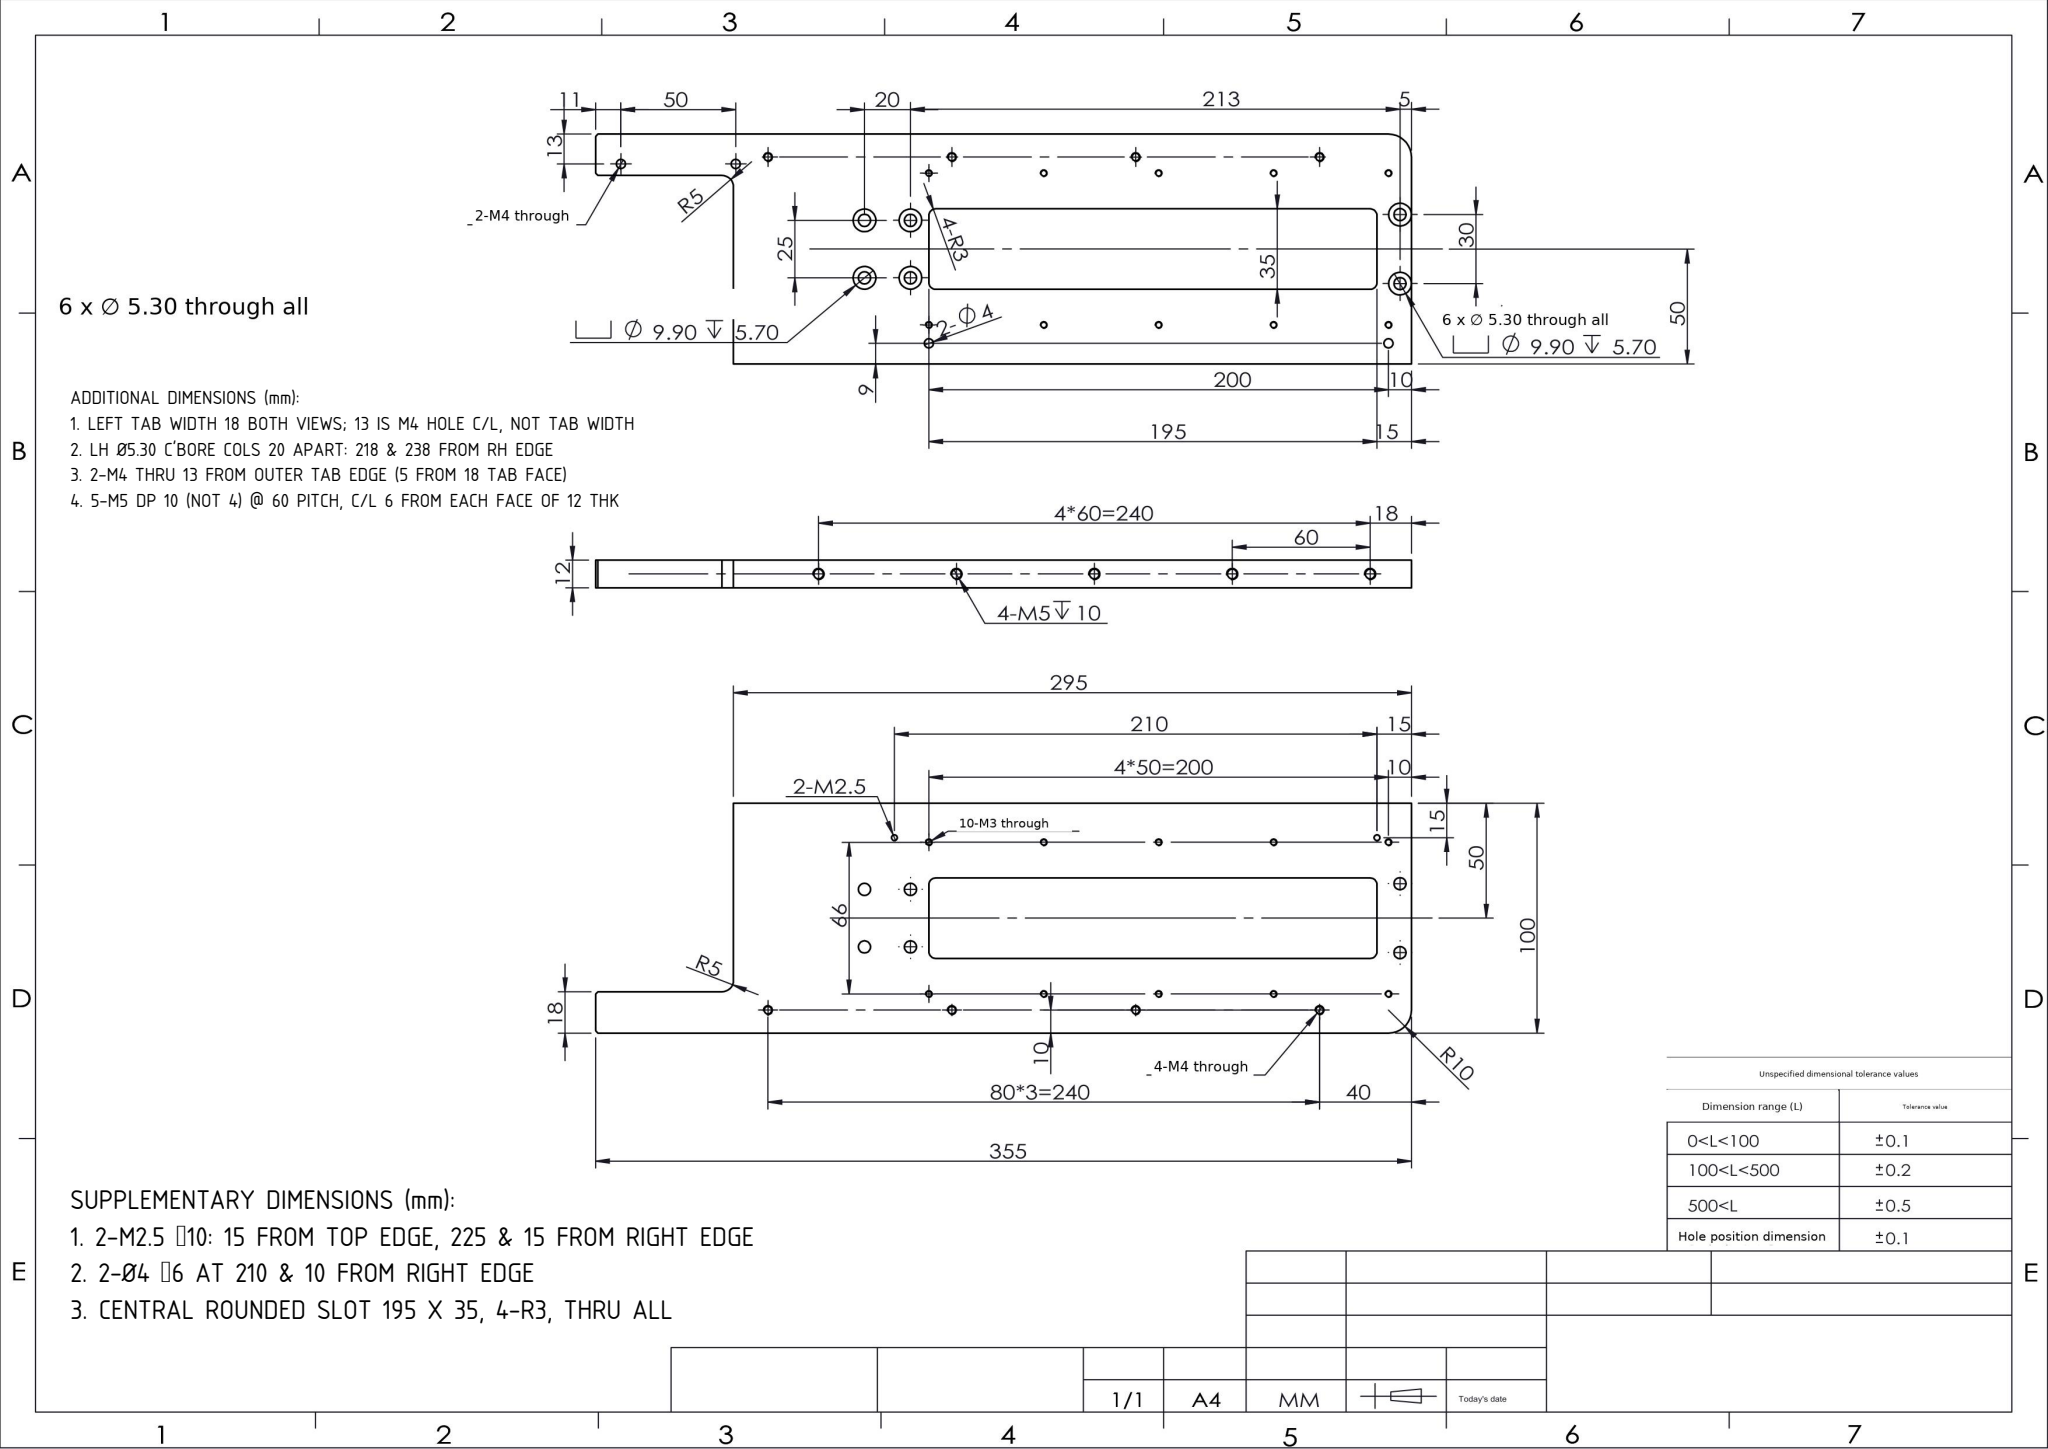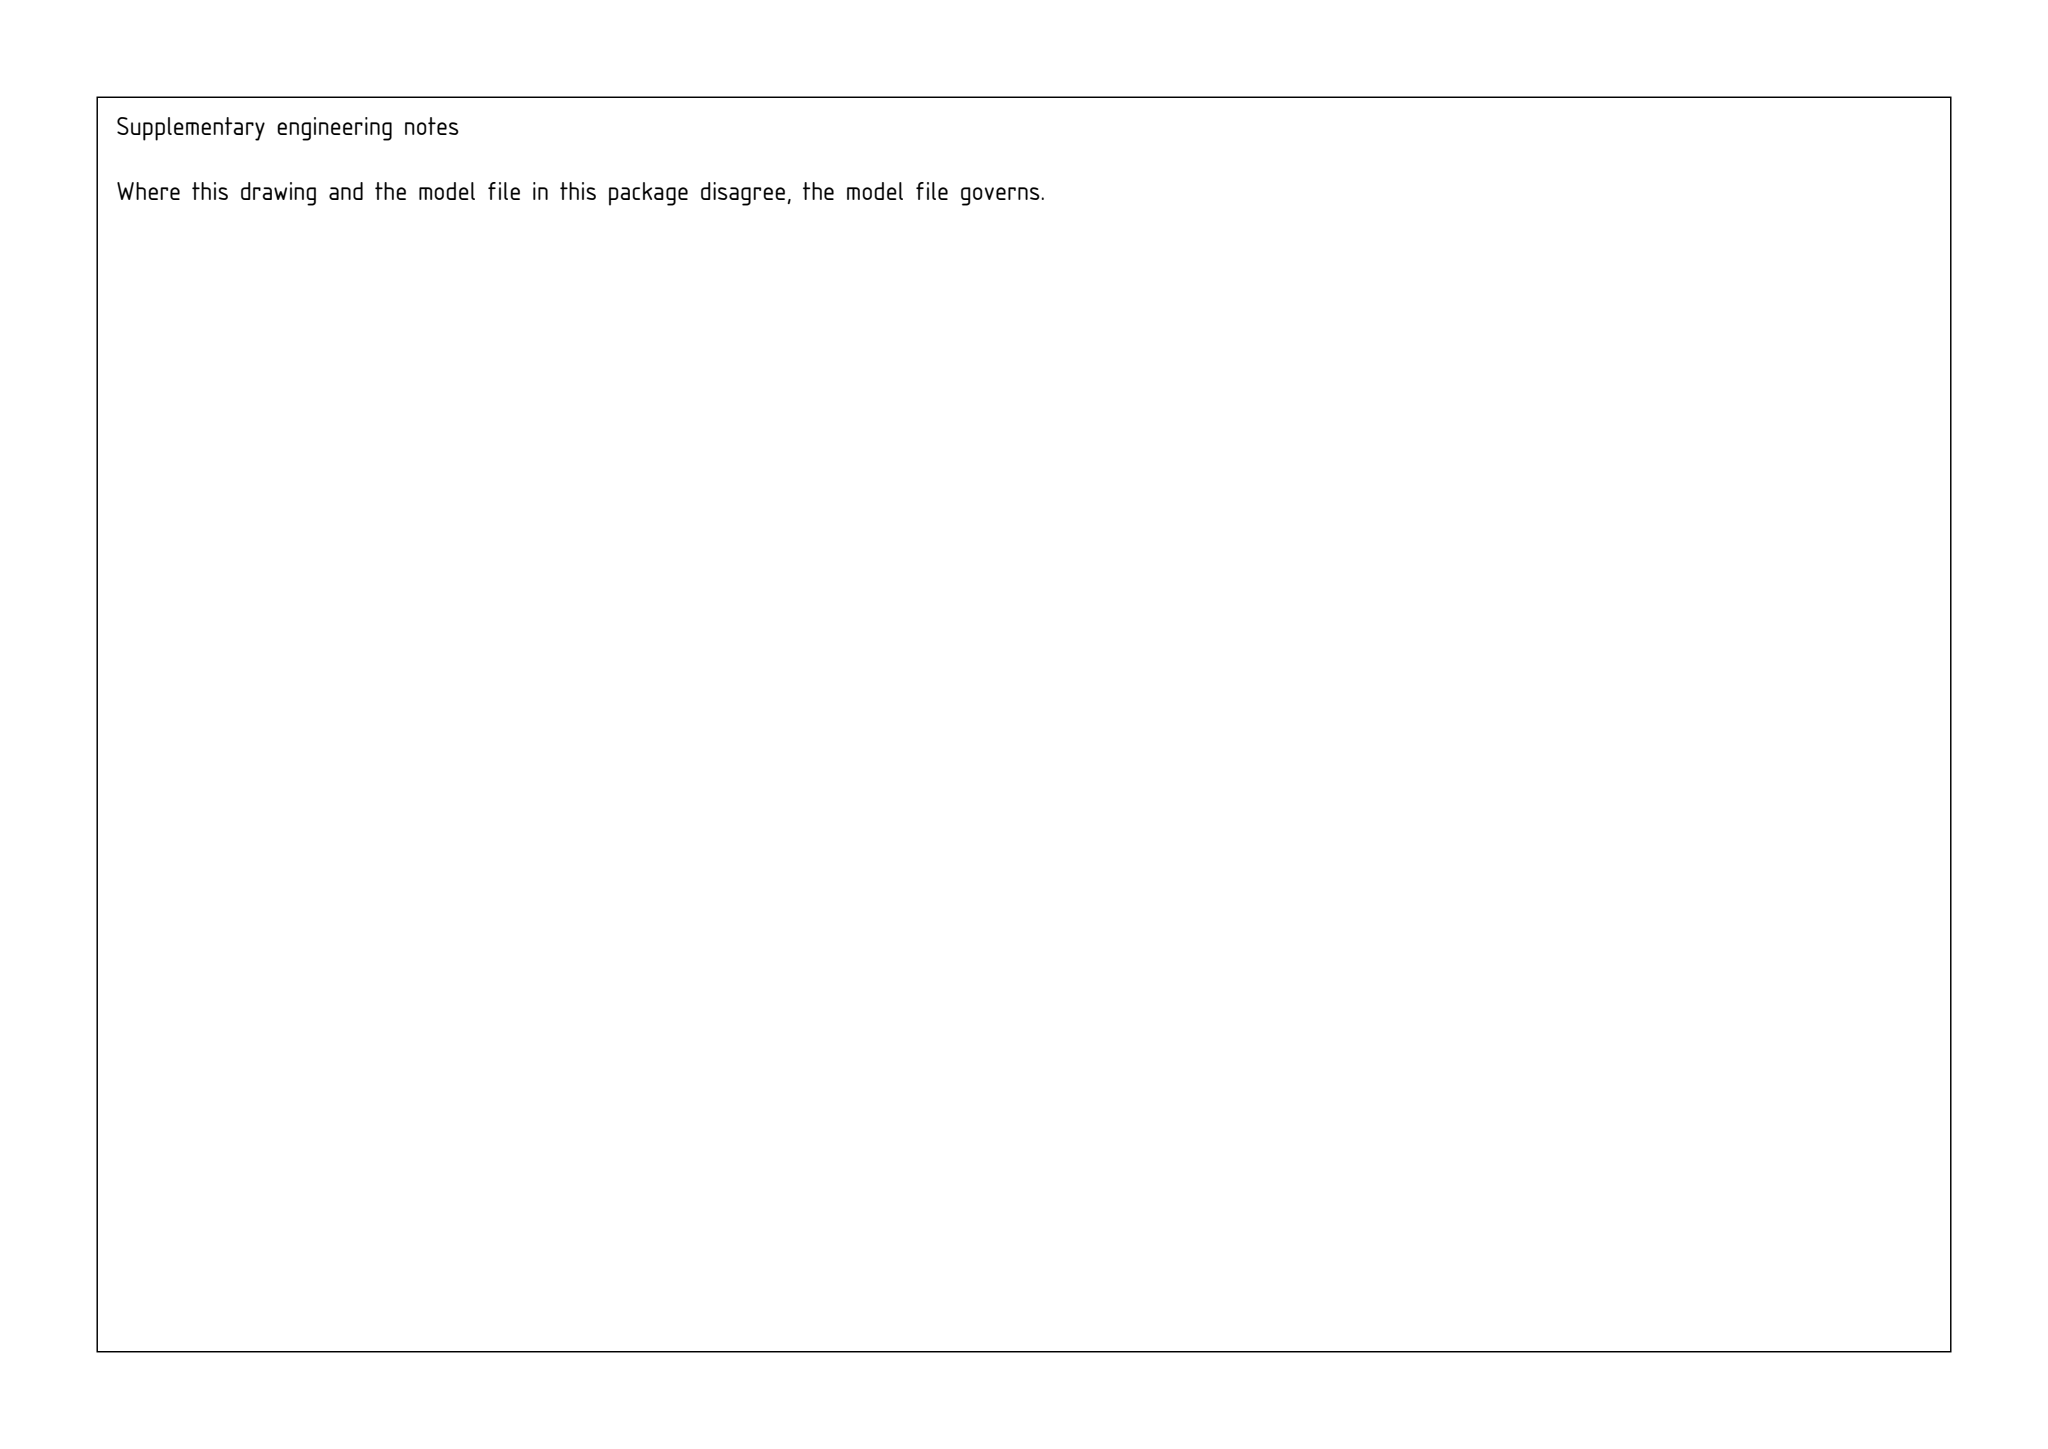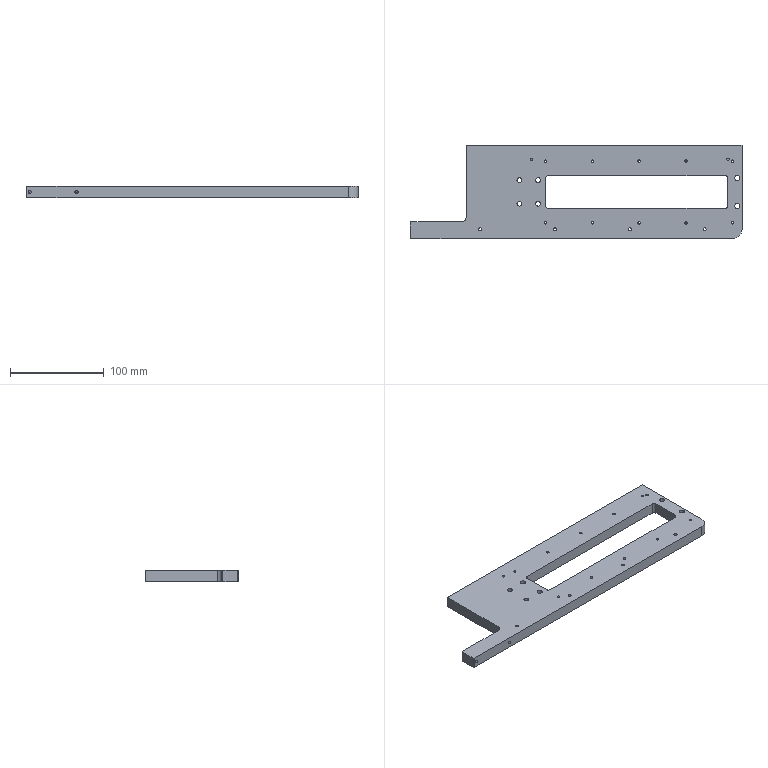Part | SolidWorks | mm | 1 solid | 124 faces | box 355 x 100 x 12 mm | volume 278915 mm3 | cylinder 84 | plane 26 | cone 14 | commonest cylinder face diameters 2.5 x24 3.3 x12 9.9 x12 5.3 x12 4.2 x10 4 x8 6 x4 10 x1
build123d program:
from build123d import *

# Parameters (mm, degrees)
BOSS_EXTRUDE1_DEPTH                                  = 12
SKETCH2_W                                            = 100
SKETCH2_H                                            = 111.825
CUT_EXTRUDE1_DEPTH                                   = 370.011
FILLET1_R                                            = 5
CHAMFER1_SIZE                                        = 1
SKETCH3_R                                            = 2
CUT_EXTRUDE2_DEPTH                                   = 10
M3_TAPPED_HOLE1_D                                    = 2.5
LPATTERN1_COUNT                                      = 5
LPATTERN1_PITCH                                      = 60
SKETCH8_W                                            = 195
SKETCH8_H                                            = 35
CUT_EXTRUDE3_DEPTH                                   = 370.011
M4_TAPPED_HOLE1_D                                    = 3.3
LPATTERN2_COUNT                                      = 4
LPATTERN2_PITCH                                      = 80
FILLET2_R                                            = 10
HOLE_SIZE_ACCORDING_TO_THE_TYPE_OF_HEXAG_D           = 5.3
HOLE_SIZE_ACCORDING_TO_THE_TYPE_OF_HEXAG_CBORE_D     = 9.9
HOLE_SIZE_ACCORDING_TO_THE_TYPE_OF_HEXAG_CBORE_DEPTH = 5.7
FILLET3_R                                            = 3
LPATTERN3_COUNT                                      = 5
LPATTERN3_PITCH                                      = 50
SKETCH23_R                                           = 1.25
CUT_EXTRUDE4_DEPTH                                   = 10
LPATTERN4_COUNT                                      = 2
LPATTERN4_PITCH                                      = 210
SKETCH24_R                                           = 2
CUT_EXTRUDE5_DEPTH                                   = 6
M4_TAPPED_HOLE2_D                                    = 3.3
M4_TAPPED_HOLE2_DEPTH                                = 10.1
M4_TAPPED_HOLE2_TIP                                  = 0.9914


with BuildPart() as part:
    # Sketch1 → Boss-Extrude1 (new body)
    with BuildSketch(Plane.XY):
        Polygon((-355, -99), (-354, -100), (0, -100), (0, 0), (-355, 0), align=None)
    extrude(amount=BOSS_EXTRUDE1_DEPTH)

    # Sketch2 → Cut-Extrude1 (cut, through all)
    with BuildSketch(Plane(origin=(0, 0, 0), x_dir=(-1, 0, 0), z_dir=(0, 0, -1))):
        with Locations((345, -26.088)):
            Rectangle(SKETCH2_W, SKETCH2_H)
    extrude(amount=-CUT_EXTRUDE1_DEPTH, mode=Mode.SUBTRACT)

    # Fillet1
    fillet1_edges = [part.edges().sort_by_distance(p)[0] for p in [
        (-295, -82, 6),
    ]]
    fillet(fillet1_edges, radius=FILLET1_R)

    # Chamfer1
    chamfer1_edges = [part.edges().sort_by_distance(p)[0] for p in [
        (-355, -82, 6),
    ]]
    chamfer(chamfer1_edges, length=CHAMFER1_SIZE)

    # Sketch3 → Cut-Extrude2 (cut)
    with BuildSketch(Plane(origin=(0, 0, 0), x_dir=(-1, 0, 0), z_dir=(0, 0, -1))):
        with Locations((344, -87)):
            Circle(SKETCH3_R)
        with Locations((294, -87)):
            Circle(SKETCH3_R)
    extrude(amount=-CUT_EXTRUDE2_DEPTH, mode=Mode.SUBTRACT)

    # Sketch4 → M5 Tapped Hole1 (revolve, cut)
    with BuildSketch(Plane(origin=(-258, 0, 6), x_dir=(0, 0, 1), z_dir=(1, 0, 0))):
        Polygon((0, 0), (0, 13.662), (2.1, 12.4), (2.1, 0), align=None)
    m5_tapped_hole1 = revolve(axis=Axis((-258, 6.35, 6), (0, -1, 0)), mode=Mode.SUBTRACT)

    # M3 Tapped Hole1 (through all)
    with Locations(Plane.XY.offset(12)):
        with Locations((-210, -17), (-210, -83)):
            m3_tapped_hole1 = Hole(M3_TAPPED_HOLE1_D / 2)

    # LPattern1: M5 Tapped Hole1 ×5
    with Locations(*[(i * LPATTERN1_PITCH, 0, 0) for i in range(1, LPATTERN1_COUNT)]):
        add(m5_tapped_hole1, mode=Mode.SUBTRACT)

    # Sketch8 → Cut-Extrude3 (cut, through all)
    with BuildSketch(Plane.XY.offset(12)):
        with Locations((-112.5, -50)):
            Rectangle(SKETCH8_W, SKETCH8_H)
    extrude(amount=-CUT_EXTRUDE3_DEPTH, mode=Mode.SUBTRACT)

    # M4 Tapped Hole1 (through all)
    with Locations(Plane(origin=(0, 0, 0), x_dir=(-1, 0, 0), z_dir=(0, 0, -1))):
        with Locations((40, -90)):
            m4_tapped_hole1 = Hole(M4_TAPPED_HOLE1_D / 2)

    # LPattern2: M4 Tapped Hole1 ×4
    with Locations(*[(-i * LPATTERN2_PITCH, 0, 0) for i in range(1, LPATTERN2_COUNT)]):
        add(m4_tapped_hole1, mode=Mode.SUBTRACT)

    # Fillet2
    fillet2_edges = [part.edges().sort_by_distance(p)[0] for p in [
        (0, -100, 6),
    ]]
    fillet(fillet2_edges, radius=FILLET2_R)

    # Hole Size according to the type of Hexag (through all)
    with Locations(Plane(origin=(0, 0, 0), x_dir=(-1, 0, 0), z_dir=(0, 0, -1))):
        with Locations((5, -65), (5, -35), (218, -62.5), (218, -37.5), (238, -37.5), (238, -62.5)):
            CounterBoreHole(HOLE_SIZE_ACCORDING_TO_THE_TYPE_OF_HEXAG_D / 2, HOLE_SIZE_ACCORDING_TO_THE_TYPE_OF_HEXAG_CBORE_D / 2, HOLE_SIZE_ACCORDING_TO_THE_TYPE_OF_HEXAG_CBORE_DEPTH)

    # Fillet3
    fillet3_edges = [part.edges().sort_by_distance(p)[0] for p in [
        (-15, -32.5, 6),
        (-15, -67.5, 6),
        (-210, -67.5, 6),
        (-210, -32.5, 6),
    ]]
    fillet(fillet3_edges, radius=FILLET3_R)

    # LPattern3: M3 Tapped Hole1 ×5
    with Locations(*[(i * LPATTERN3_PITCH, 0, 0) for i in range(1, LPATTERN3_COUNT)]):
        add(m3_tapped_hole1, mode=Mode.SUBTRACT)

    # Sketch23 → Cut-Extrude4 (cut)
    with BuildSketch(Plane.XY.offset(12)):
        with Locations((-15, -15)):
            Circle(SKETCH23_R)
    cut_extrude4 = extrude(amount=-CUT_EXTRUDE4_DEPTH, mode=Mode.SUBTRACT)

    # LPattern4: Cut-Extrude4 ×2
    with Locations(*[(-i * LPATTERN4_PITCH, 0, 0) for i in range(1, LPATTERN4_COUNT)]):
        add(cut_extrude4, mode=Mode.SUBTRACT)

    # Sketch24 → Cut-Extrude5 (cut)
    with BuildSketch(Plane(origin=(0, 0, 0), x_dir=(-1, 0, 0), z_dir=(0, 0, -1))):
        with Locations((210, -9)):
            Circle(SKETCH24_R)
        with Locations((10, -9)):
            Circle(SKETCH24_R)
    extrude(amount=-CUT_EXTRUDE5_DEPTH, mode=Mode.SUBTRACT)

    # M4 Tapped Hole2
    with Locations(Plane(origin=(0, -100, 0), x_dir=(-1, 0, 0), z_dir=(0, -1, 0))):
        with Locations((351, -6), (301, -6)):
            Hole(M4_TAPPED_HOLE2_D / 2, depth=M4_TAPPED_HOLE2_DEPTH)
            with Locations((0, 0, -(M4_TAPPED_HOLE2_DEPTH + M4_TAPPED_HOLE2_TIP / 2))):  # 118° drill point
                Cone(0, M4_TAPPED_HOLE2_D / 2, M4_TAPPED_HOLE2_TIP, mode=Mode.SUBTRACT)


solid = part.part